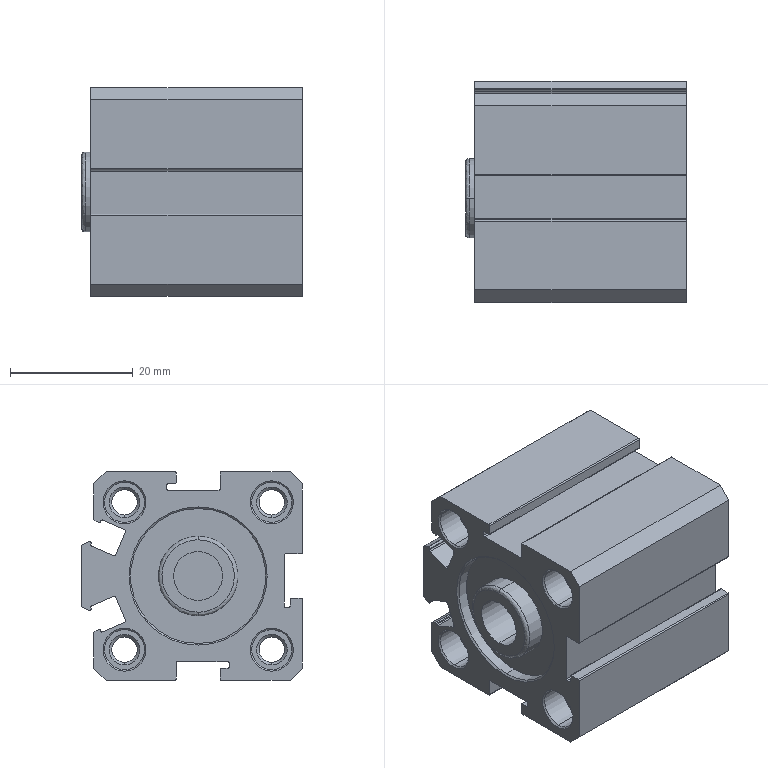Component | SolidWorks | Ultra-thinCylinderSDA2015-1_SDA2015Cylinder-1 | 1 solid | 215 faces | volume 25973 mm3 | cylinder 90 | plane 67 | cone 56 | spline 2 | commonest cylinder face diameters 0.4 x26 4.134 x20 6.5 x16 4.2 x8 0.8 x5 0.6 x5 20 x4 22 x2